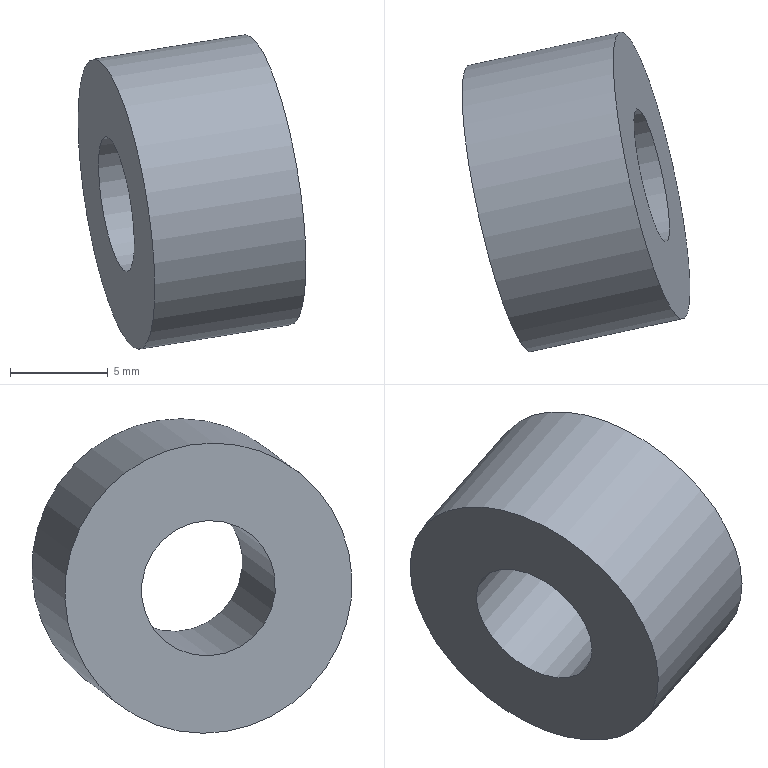Component | NX | 4 | 1 solid | 4 faces | box 11.64 x 16.35 x 16.06 mm | volume 1106 mm3 | cylinder 2 | plane 2 | commonest cylinder face diameters 15 x1 7 x1
STEP:
#1=CARTESIAN_POINT('',(0.,0.,0.));
#2=DIRECTION('',(0.,0.,1.));
#3=DIRECTION('',(1.,0.,0.));
#4=AXIS2_PLACEMENT_3D('',#1,#2,#3);
#5=CARTESIAN_POINT('',(56.127,515.263,-180.707));
#6=VERTEX_POINT('',#5);
#7=CARTESIAN_POINT('',(55.113,522.091,-183.639));
#8=DIRECTION('',(0.9653,0.21,0.1554));
#9=DIRECTION('',(0.1351,-0.9104,0.3909));
#10=AXIS2_PLACEMENT_3D('',#7,#8,#9);
#11=CIRCLE('',#10,7.5);
#12=CARTESIAN_POINT('',(55.113,522.091,-183.639));
#13=DIRECTION('',(0.9653,0.21,0.1554));
#14=DIRECTION('',(-0.2236,0.3563,0.9072));
#15=AXIS2_PLACEMENT_3D('',#12,#13,#14);
#16=CYLINDRICAL_SURFACE('',#15,7.5);
#17=CARTESIAN_POINT('',(1.571,0.));
#18=DIRECTION('',(1.,0.));
#19=VECTOR('',#18,1.);
#20=LINE('',#17,#19);
#21=(GEOMETRIC_REPRESENTATION_CONTEXT(2)PARAMETRIC_REPRESENTATION_CONTEXT()REPRESENTATION_CONTEXT('',''));
#22=DEFINITIONAL_REPRESENTATION('',(#20),#21);
#23=PCURVE('',#16,#22);
#24=CARTESIAN_POINT('',(55.113,522.091,-183.639));
#25=DIRECTION('',(0.9653,0.21,0.1554));
#26=DIRECTION('',(-0.2236,0.3563,0.9072));
#27=AXIS2_PLACEMENT_3D('',#24,#25,#26);
#28=PLANE('',#27);
#29=CARTESIAN_POINT('',(0.,0.));
#30=DIRECTION('',(-0.,1.));
#31=AXIS2_PLACEMENT_2D('',#29,#30);
#32=CIRCLE('',#31,7.5);
#33=(GEOMETRIC_REPRESENTATION_CONTEXT(2)PARAMETRIC_REPRESENTATION_CONTEXT()REPRESENTATION_CONTEXT('',''));
#34=DEFINITIONAL_REPRESENTATION('',(#32),#33);
#35=PCURVE('',#28,#34);
#36=SURFACE_CURVE('',#11,(#23,#35),.PCURVE_S1.);
#37=EDGE_CURVE('',#6,#6,#36,.T.);
#38=ORIENTED_EDGE('',*,*,#37,.T.);
#39=CARTESIAN_POINT('',(63.849,516.943,-179.463));
#40=VERTEX_POINT('',#39);
#41=CARTESIAN_POINT('',(56.127,515.263,-180.707));
#42=CARTESIAN_POINT('',(63.849,516.943,-179.463));
#43=B_SPLINE_CURVE_WITH_KNOTS('',1,(#41,#42),.UNSPECIFIED.,.F.,.F.,(2,2),(0.,8.),.PIECEWISE_BEZIER_KNOTS.);
#44=CARTESIAN_POINT('',(7.854,0.));
#45=DIRECTION('',(0.,1.));
#46=VECTOR('',#45,1.);
#47=LINE('',#44,#46);
#48=(GEOMETRIC_REPRESENTATION_CONTEXT(2)PARAMETRIC_REPRESENTATION_CONTEXT()REPRESENTATION_CONTEXT('',''));
#49=DEFINITIONAL_REPRESENTATION('',(#47),#48);
#50=PCURVE('',#16,#49);
#51=CARTESIAN_POINT('',(1.571,0.));
#52=DIRECTION('',(0.,1.));
#53=VECTOR('',#52,1.);
#54=LINE('',#51,#53);
#55=(GEOMETRIC_REPRESENTATION_CONTEXT(2)PARAMETRIC_REPRESENTATION_CONTEXT()REPRESENTATION_CONTEXT('',''));
#56=DEFINITIONAL_REPRESENTATION('',(#54),#55);
#57=PCURVE('',#16,#56);
#58=SEAM_CURVE('',#43,(#50,#57),.PCURVE_S1.);
#59=EDGE_CURVE('',#6,#40,#58,.T.);
#60=ORIENTED_EDGE('',*,*,#59,.T.);
#61=CARTESIAN_POINT('',(62.835,523.771,-182.395));
#62=DIRECTION('',(0.9653,0.21,0.1554));
#63=DIRECTION('',(0.1351,-0.9104,0.3909));
#64=AXIS2_PLACEMENT_3D('',#61,#62,#63);
#65=CIRCLE('',#64,7.5);
#66=CARTESIAN_POINT('',(1.571,8.));
#67=DIRECTION('',(1.,0.));
#68=VECTOR('',#67,1.);
#69=LINE('',#66,#68);
#70=(GEOMETRIC_REPRESENTATION_CONTEXT(2)PARAMETRIC_REPRESENTATION_CONTEXT()REPRESENTATION_CONTEXT('',''));
#71=DEFINITIONAL_REPRESENTATION('',(#69),#70);
#72=PCURVE('',#16,#71);
#73=CARTESIAN_POINT('',(62.835,523.771,-182.395));
#74=DIRECTION('',(0.9653,0.21,0.1554));
#75=DIRECTION('',(-0.2236,0.3563,0.9072));
#76=AXIS2_PLACEMENT_3D('',#73,#74,#75);
#77=PLANE('',#76);
#78=CARTESIAN_POINT('',(0.,0.));
#79=DIRECTION('',(-0.,1.));
#80=AXIS2_PLACEMENT_2D('',#78,#79);
#81=CIRCLE('',#80,7.5);
#82=(GEOMETRIC_REPRESENTATION_CONTEXT(2)PARAMETRIC_REPRESENTATION_CONTEXT()REPRESENTATION_CONTEXT('',''));
#83=DEFINITIONAL_REPRESENTATION('',(#81),#82);
#84=PCURVE('',#77,#83);
#85=SURFACE_CURVE('',#65,(#72,#84),.PCURVE_S1.);
#86=EDGE_CURVE('',#40,#40,#85,.T.);
#87=ORIENTED_EDGE('',*,*,#86,.F.);
#88=ORIENTED_EDGE('',*,*,#59,.F.);
#89=EDGE_LOOP('',(#38,#60,#87,#88));
#90=FACE_BOUND('',#89,.T.);
#91=ADVANCED_FACE('',(#90),#16,.T.);
#92=CARTESIAN_POINT('',(55.586,518.905,-182.271));
#93=VERTEX_POINT('',#92);
#94=CARTESIAN_POINT('',(55.113,522.091,-183.639));
#95=DIRECTION('',(0.9653,0.21,0.1554));
#96=DIRECTION('',(0.1351,-0.9104,0.3909));
#97=AXIS2_PLACEMENT_3D('',#94,#95,#96);
#98=CIRCLE('',#97,3.5);
#99=CARTESIAN_POINT('',(55.113,522.091,-183.639));
#100=DIRECTION('',(0.9653,0.21,0.1554));
#101=DIRECTION('',(-0.2236,0.3563,0.9072));
#102=AXIS2_PLACEMENT_3D('',#99,#100,#101);
#103=CYLINDRICAL_SURFACE('',#102,3.5);
#104=CARTESIAN_POINT('',(1.571,0.));
#105=DIRECTION('',(1.,0.));
#106=VECTOR('',#105,1.);
#107=LINE('',#104,#106);
#108=(GEOMETRIC_REPRESENTATION_CONTEXT(2)PARAMETRIC_REPRESENTATION_CONTEXT()REPRESENTATION_CONTEXT('',''));
#109=DEFINITIONAL_REPRESENTATION('',(#107),#108);
#110=PCURVE('',#103,#109);
#111=CARTESIAN_POINT('',(0.,0.));
#112=DIRECTION('',(0.,1.));
#113=AXIS2_PLACEMENT_2D('',#111,#112);
#114=CIRCLE('',#113,3.5);
#115=(GEOMETRIC_REPRESENTATION_CONTEXT(2)PARAMETRIC_REPRESENTATION_CONTEXT()REPRESENTATION_CONTEXT('',''));
#116=DEFINITIONAL_REPRESENTATION('',(#114),#115);
#117=PCURVE('',#28,#116);
#118=SURFACE_CURVE('',#98,(#110,#117),.PCURVE_S1.);
#119=EDGE_CURVE('',#93,#93,#118,.T.);
#120=ORIENTED_EDGE('',*,*,#119,.T.);
#121=CARTESIAN_POINT('',(63.308,520.585,-181.027));
#122=VERTEX_POINT('',#121);
#123=CARTESIAN_POINT('',(55.586,518.905,-182.271));
#124=CARTESIAN_POINT('',(63.308,520.585,-181.027));
#125=B_SPLINE_CURVE_WITH_KNOTS('',1,(#123,#124),.UNSPECIFIED.,.F.,.F.,(2,2),(0.,8.),.PIECEWISE_BEZIER_KNOTS.);
#126=CARTESIAN_POINT('',(7.854,0.));
#127=DIRECTION('',(0.,1.));
#128=VECTOR('',#127,1.);
#129=LINE('',#126,#128);
#130=(GEOMETRIC_REPRESENTATION_CONTEXT(2)PARAMETRIC_REPRESENTATION_CONTEXT()REPRESENTATION_CONTEXT('',''));
#131=DEFINITIONAL_REPRESENTATION('',(#129),#130);
#132=PCURVE('',#103,#131);
#133=CARTESIAN_POINT('',(1.571,0.));
#134=DIRECTION('',(0.,1.));
#135=VECTOR('',#134,1.);
#136=LINE('',#133,#135);
#137=(GEOMETRIC_REPRESENTATION_CONTEXT(2)PARAMETRIC_REPRESENTATION_CONTEXT()REPRESENTATION_CONTEXT('',''));
#138=DEFINITIONAL_REPRESENTATION('',(#136),#137);
#139=PCURVE('',#103,#138);
#140=SEAM_CURVE('',#125,(#132,#139),.PCURVE_S1.);
#141=EDGE_CURVE('',#93,#122,#140,.T.);
#142=ORIENTED_EDGE('',*,*,#141,.T.);
#143=CARTESIAN_POINT('',(62.835,523.771,-182.395));
#144=DIRECTION('',(0.9653,0.21,0.1554));
#145=DIRECTION('',(0.1351,-0.9104,0.3909));
#146=AXIS2_PLACEMENT_3D('',#143,#144,#145);
#147=CIRCLE('',#146,3.5);
#148=CARTESIAN_POINT('',(1.571,8.));
#149=DIRECTION('',(1.,0.));
#150=VECTOR('',#149,1.);
#151=LINE('',#148,#150);
#152=(GEOMETRIC_REPRESENTATION_CONTEXT(2)PARAMETRIC_REPRESENTATION_CONTEXT()REPRESENTATION_CONTEXT('',''));
#153=DEFINITIONAL_REPRESENTATION('',(#151),#152);
#154=PCURVE('',#103,#153);
#155=CARTESIAN_POINT('',(0.,0.));
#156=DIRECTION('',(0.,1.));
#157=AXIS2_PLACEMENT_2D('',#155,#156);
#158=CIRCLE('',#157,3.5);
#159=(GEOMETRIC_REPRESENTATION_CONTEXT(2)PARAMETRIC_REPRESENTATION_CONTEXT()REPRESENTATION_CONTEXT('',''));
#160=DEFINITIONAL_REPRESENTATION('',(#158),#159);
#161=PCURVE('',#77,#160);
#162=SURFACE_CURVE('',#147,(#154,#161),.PCURVE_S1.);
#163=EDGE_CURVE('',#122,#122,#162,.T.);
#164=ORIENTED_EDGE('',*,*,#163,.F.);
#165=ORIENTED_EDGE('',*,*,#141,.F.);
#166=EDGE_LOOP('',(#120,#142,#164,#165));
#167=FACE_BOUND('',#166,.F.);
#168=ADVANCED_FACE('',(#167),#103,.F.);
#169=ORIENTED_EDGE('',*,*,#37,.F.);
#170=EDGE_LOOP('',(#169));
#171=FACE_BOUND('',#170,.T.);
#172=ORIENTED_EDGE('',*,*,#119,.T.);
#173=EDGE_LOOP('',(#172));
#174=FACE_BOUND('',#173,.T.);
#175=ADVANCED_FACE('',(#171,#174),#28,.F.);
#176=ORIENTED_EDGE('',*,*,#86,.T.);
#177=EDGE_LOOP('',(#176));
#178=FACE_BOUND('',#177,.T.);
#179=ORIENTED_EDGE('',*,*,#163,.F.);
#180=EDGE_LOOP('',(#179));
#181=FACE_BOUND('',#180,.T.);
#182=ADVANCED_FACE('',(#178,#181),#77,.T.);
#183=CLOSED_SHELL('',(#91,#168,#175,#182));
#184=MANIFOLD_SOLID_BREP('',#183);
#185=(LENGTH_UNIT()NAMED_UNIT(*)SI_UNIT(.MILLI.,.METRE.));
#186=UNCERTAINTY_MEASURE_WITH_UNIT(LENGTH_MEASURE(0.00001),#185,'','');
#187=(NAMED_UNIT(*)PLANE_ANGLE_UNIT()SI_UNIT($,.RADIAN.));
#188=(NAMED_UNIT(*)SI_UNIT($,.STERADIAN.)SOLID_ANGLE_UNIT());
#189=(GEOMETRIC_REPRESENTATION_CONTEXT(3)GLOBAL_UNCERTAINTY_ASSIGNED_CONTEXT((#186))GLOBAL_UNIT_ASSIGNED_CONTEXT((#185,#187,#188))REPRESENTATION_CONTEXT('',''));
#190=ADVANCED_BREP_SHAPE_REPRESENTATION('',(#4,#184),#189);